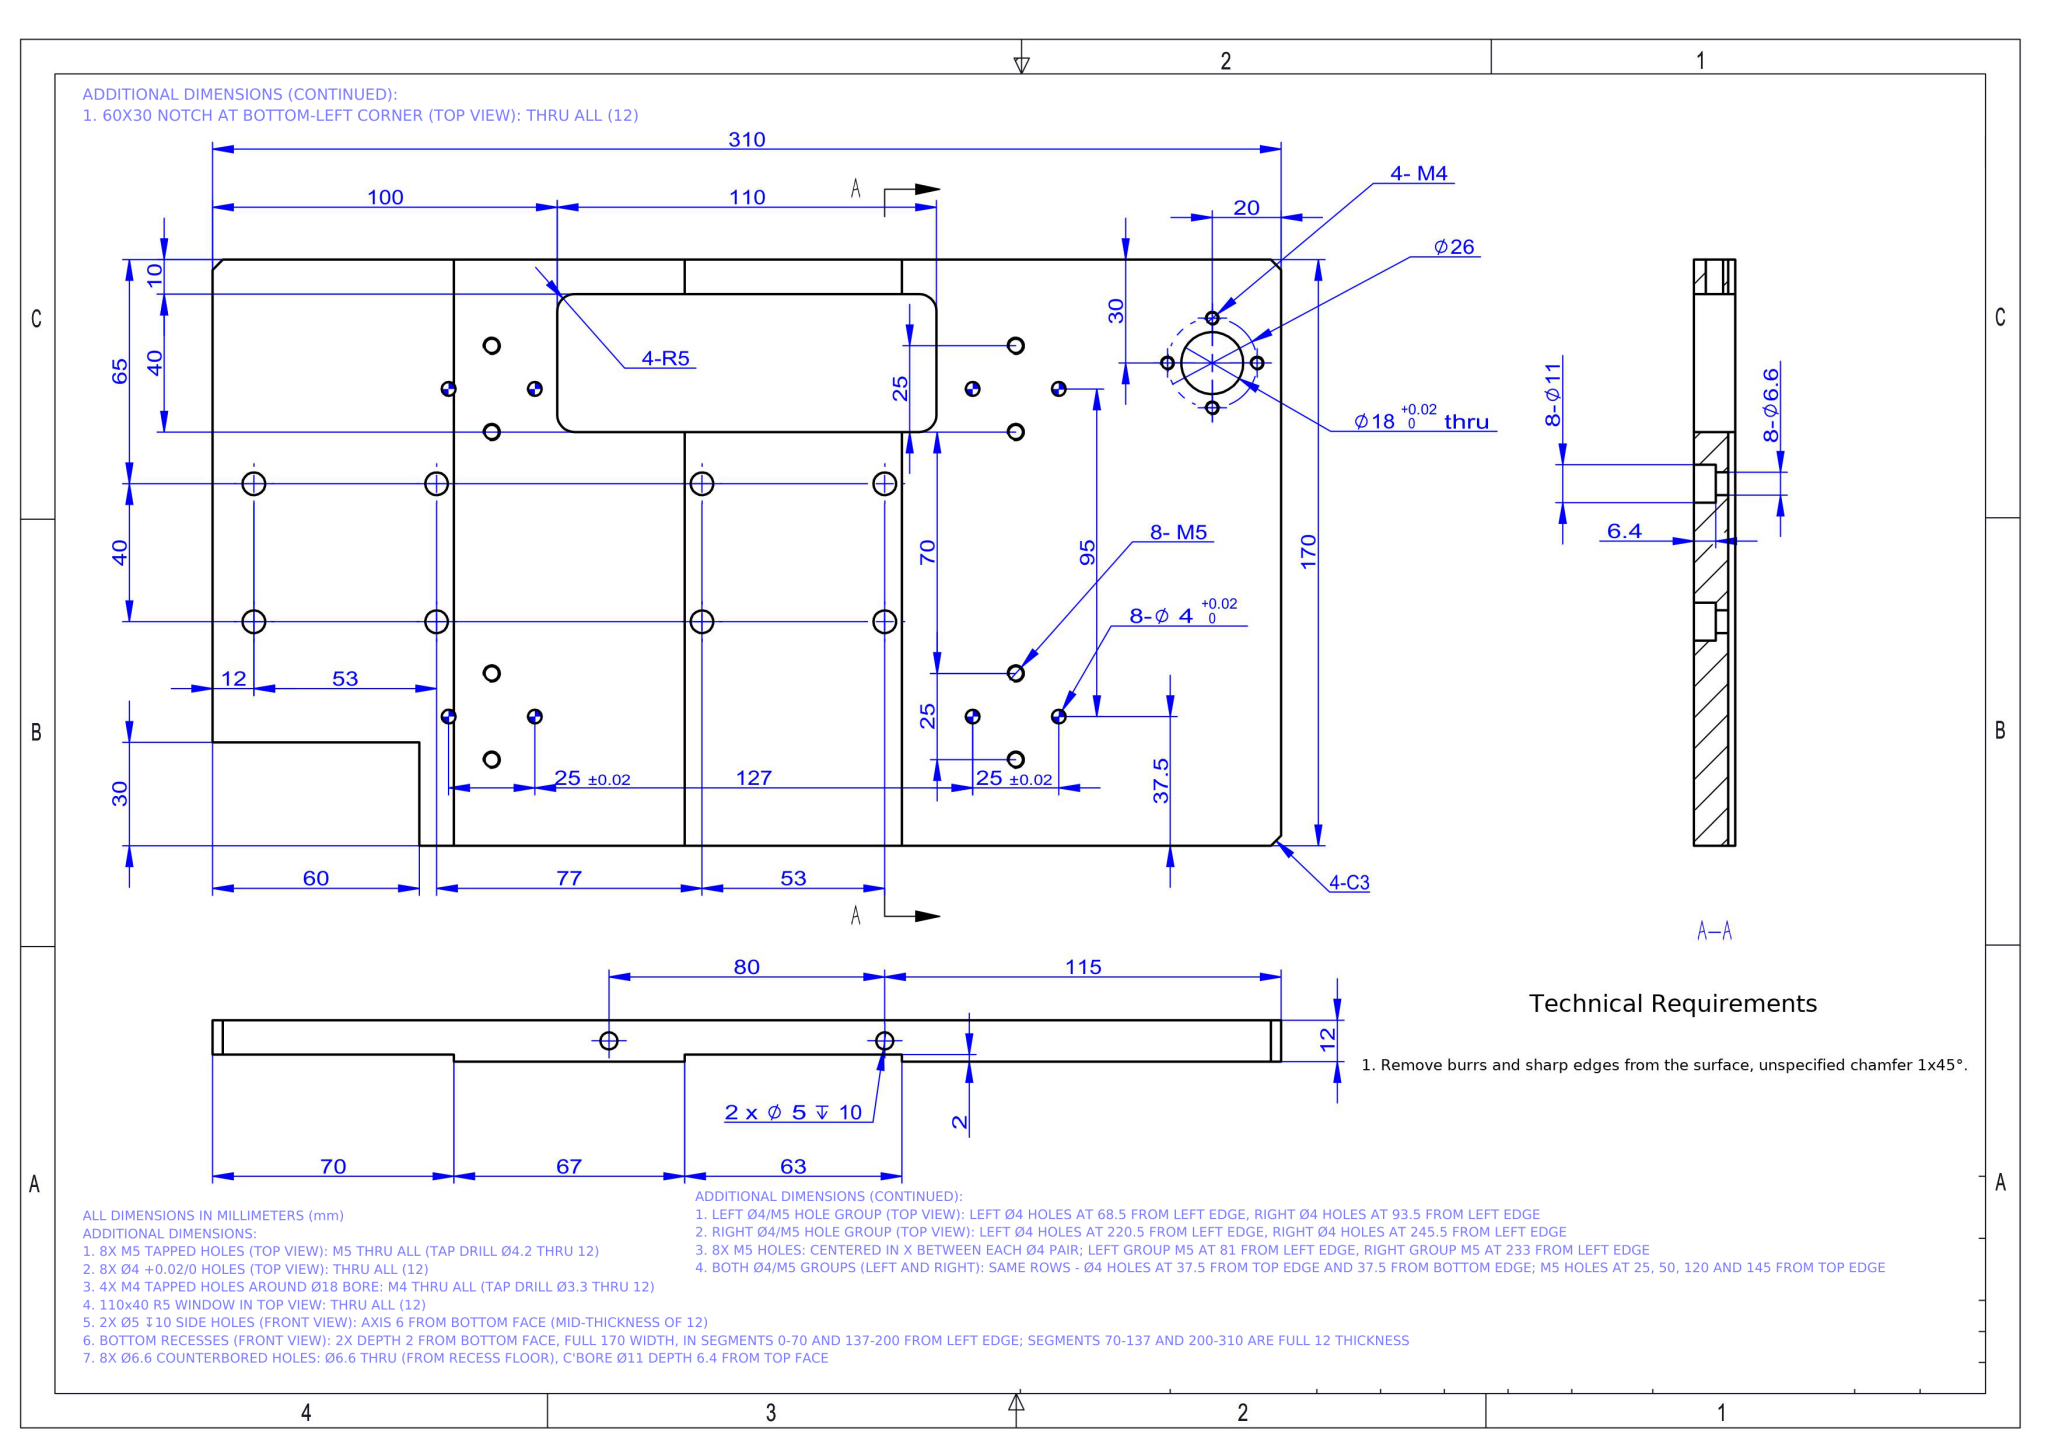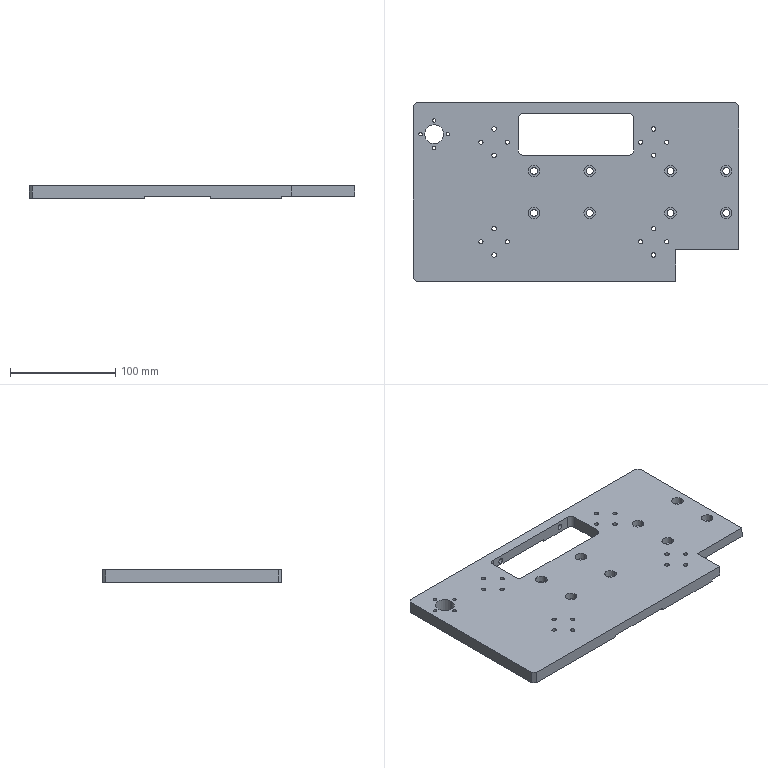Part | NX | mm | 1 solid | 116 faces | box 310 x 170 x 12 mm | volume 509327 mm3 | cylinder 82 | plane 34 | commonest cylinder face diameters 4.2 x16 4 x16 11 x16 6.6 x16 3.3 x8 5 x4 10 x4 18 x2